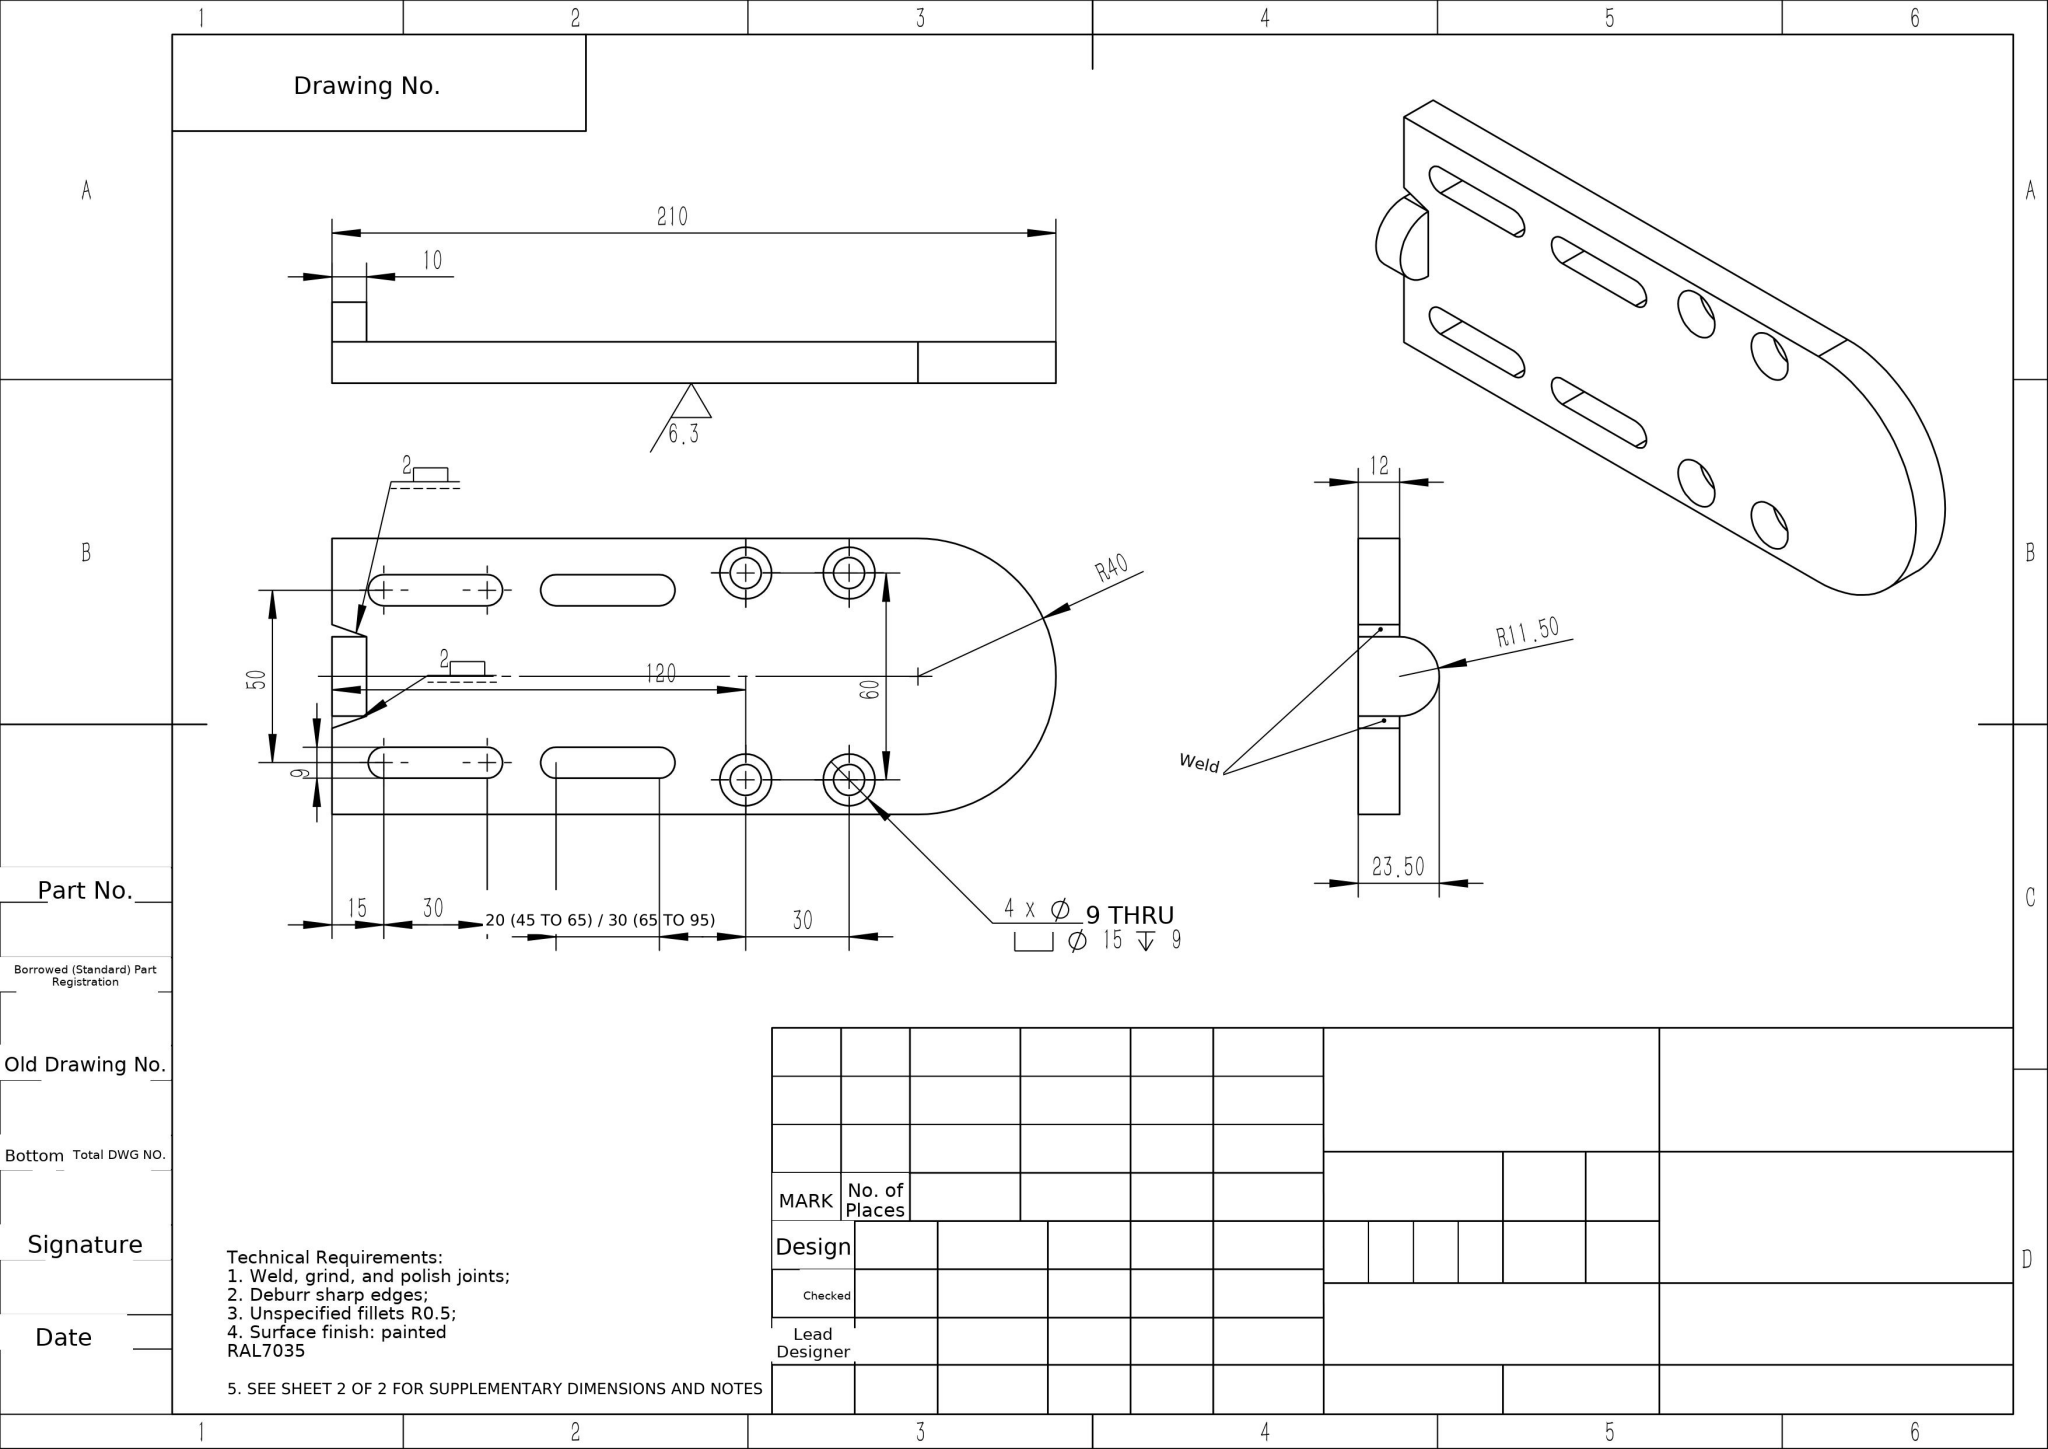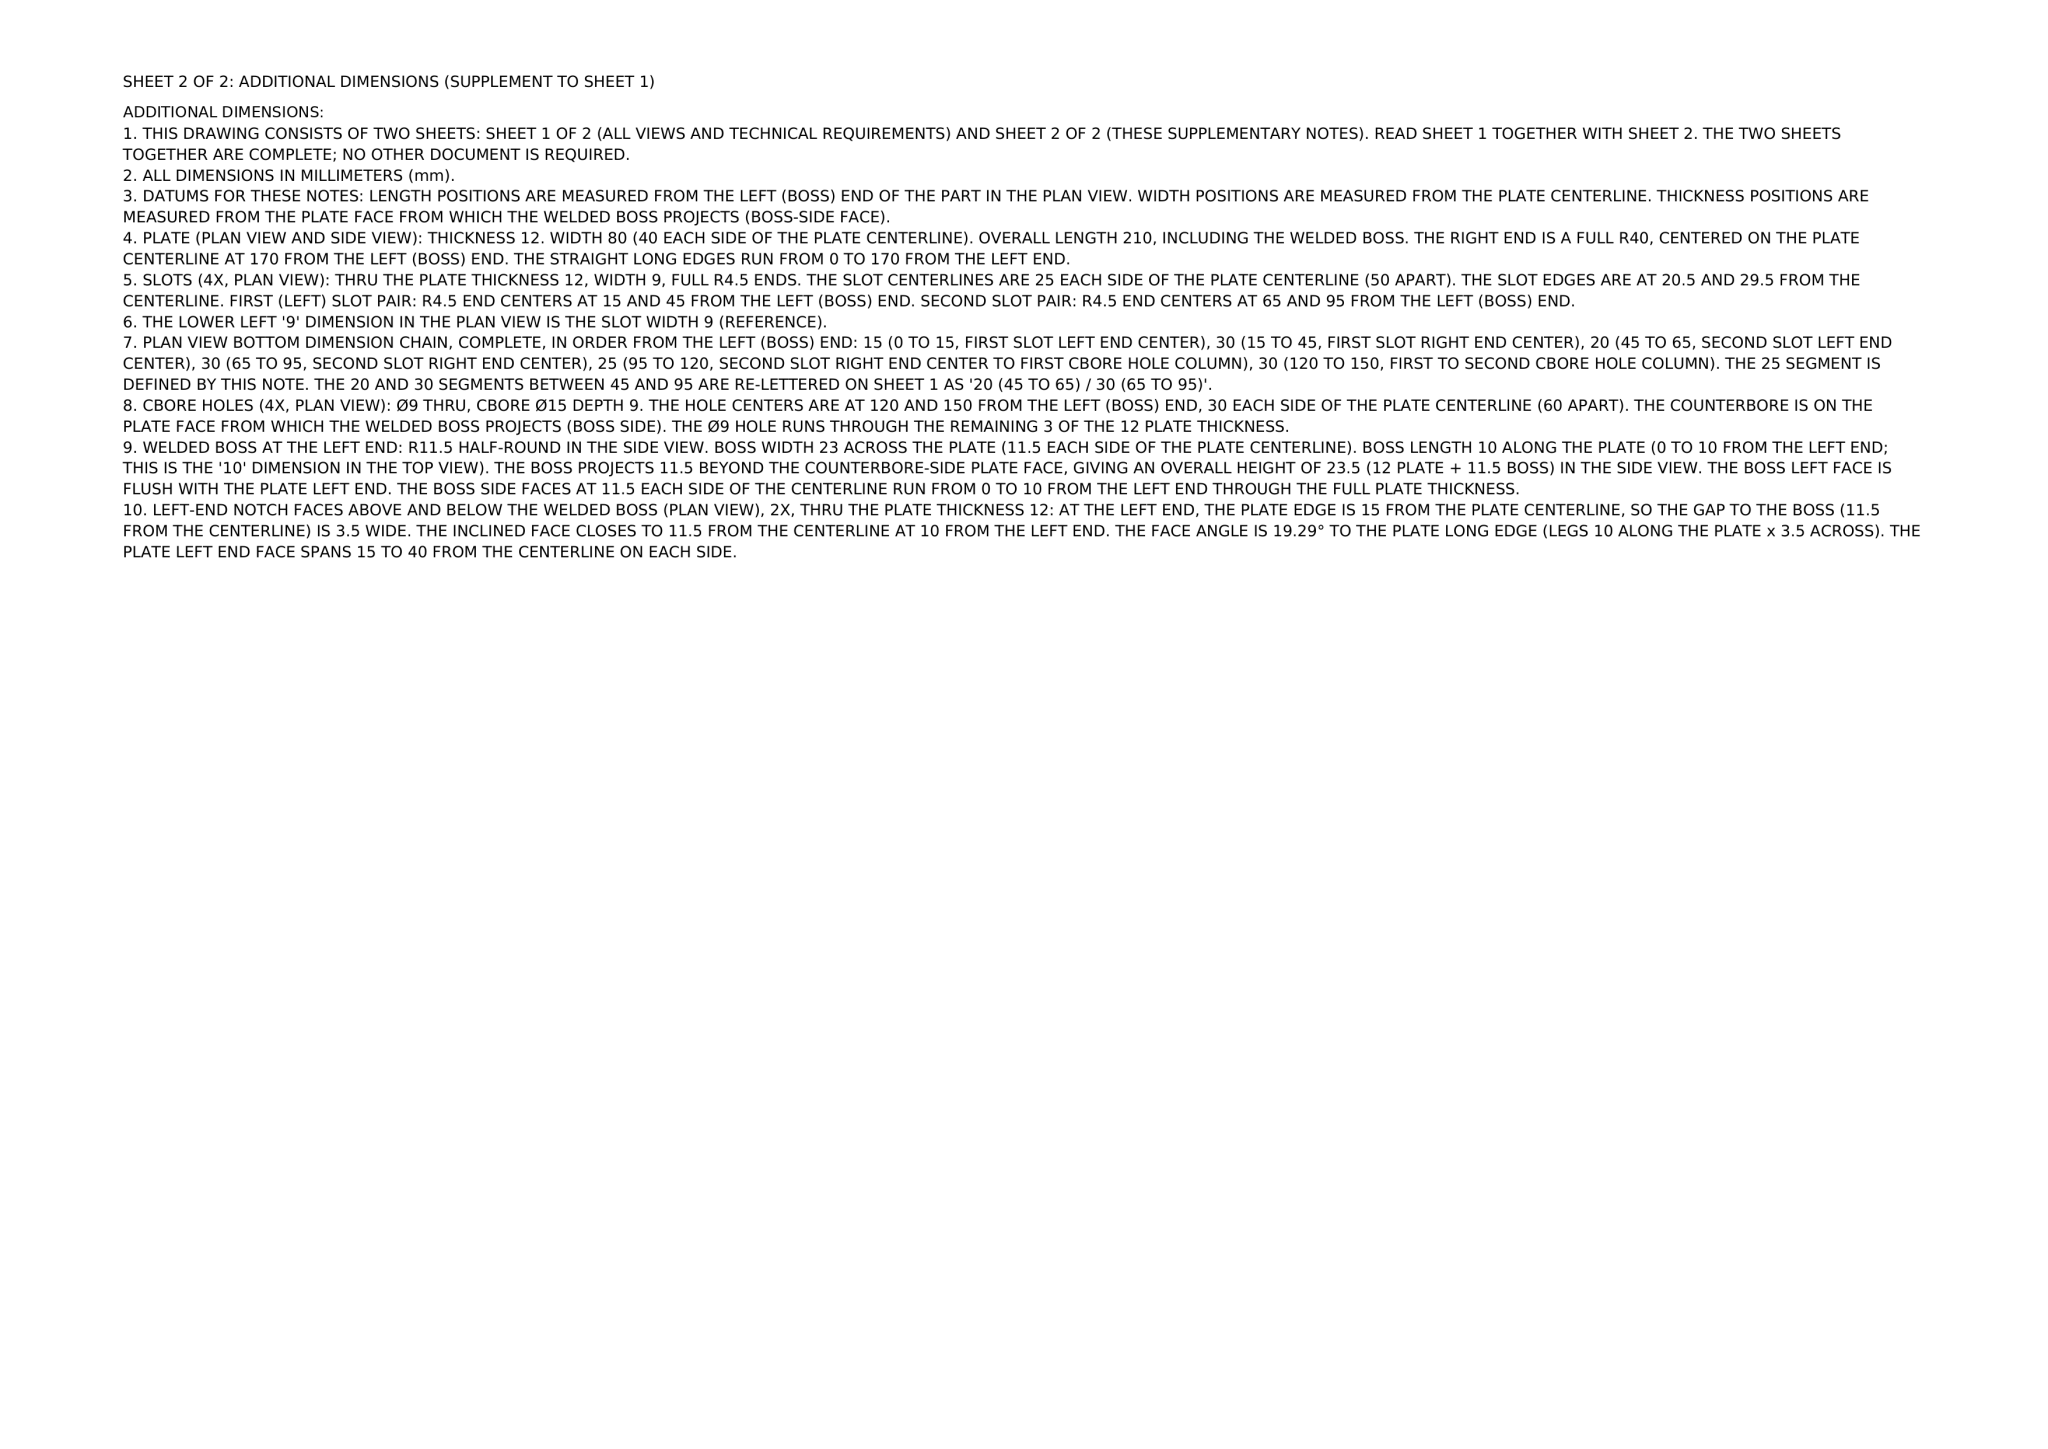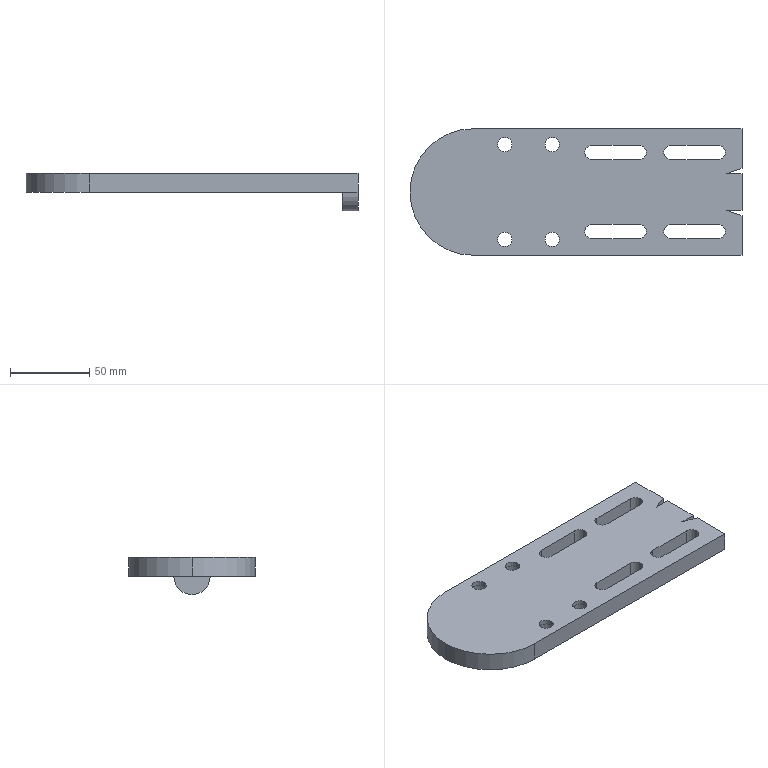Part | NX | mm | 1 solid | 55 faces | box 210 x 80 x 23.5 mm | volume 171878 mm3 | cylinder 31 | plane 24 | commonest cylinder face diameters 9 x20 15 x8 80 x2 23 x1